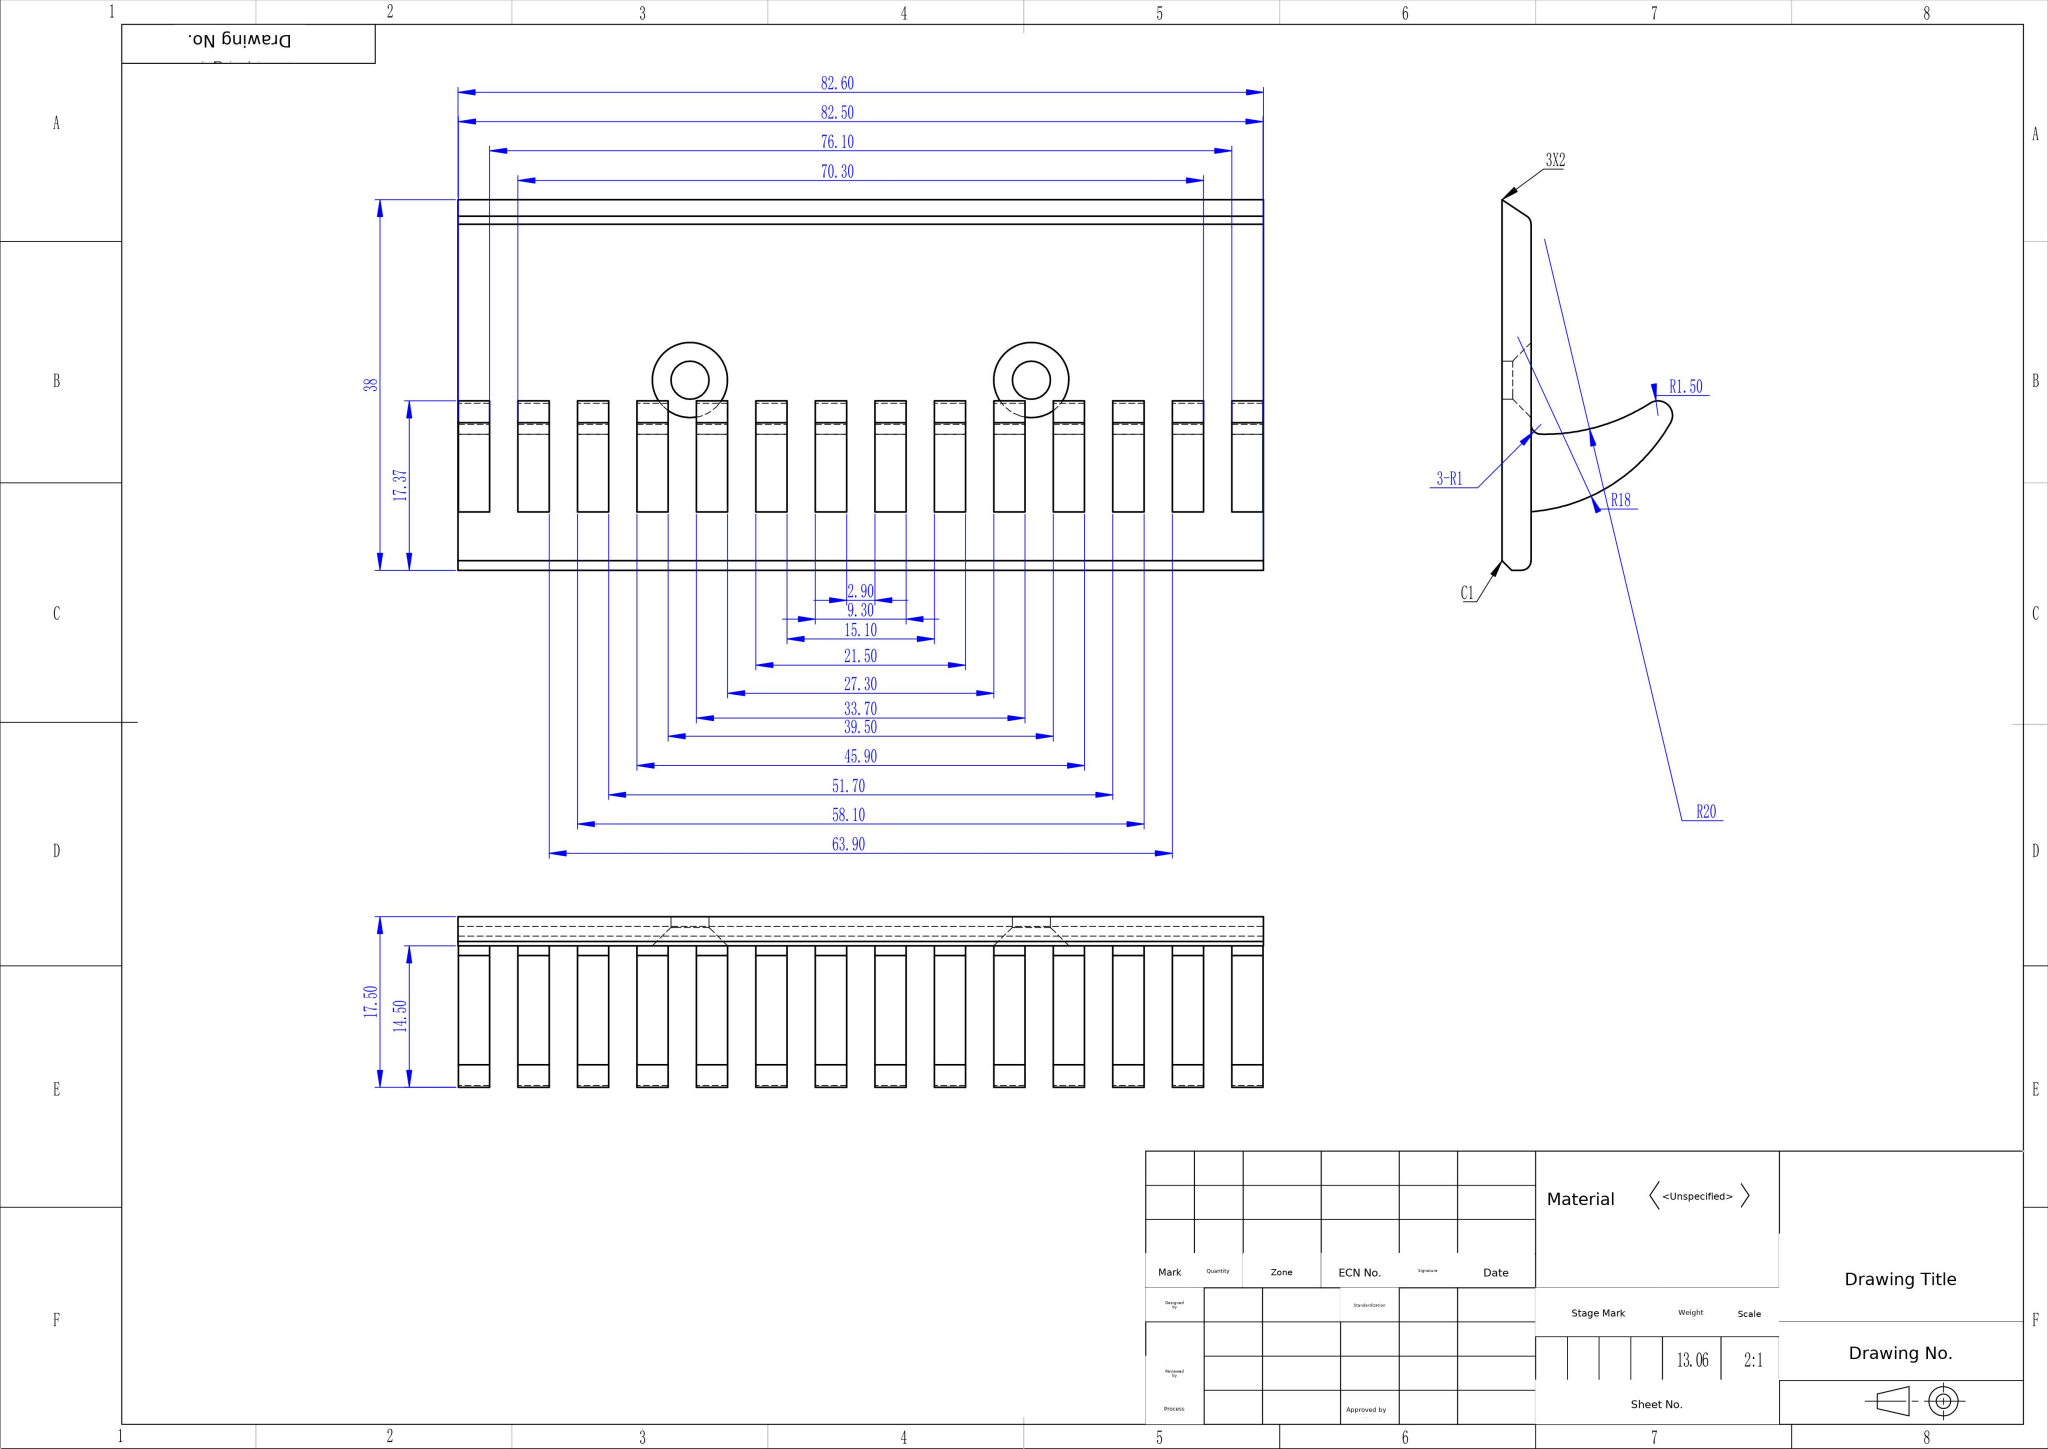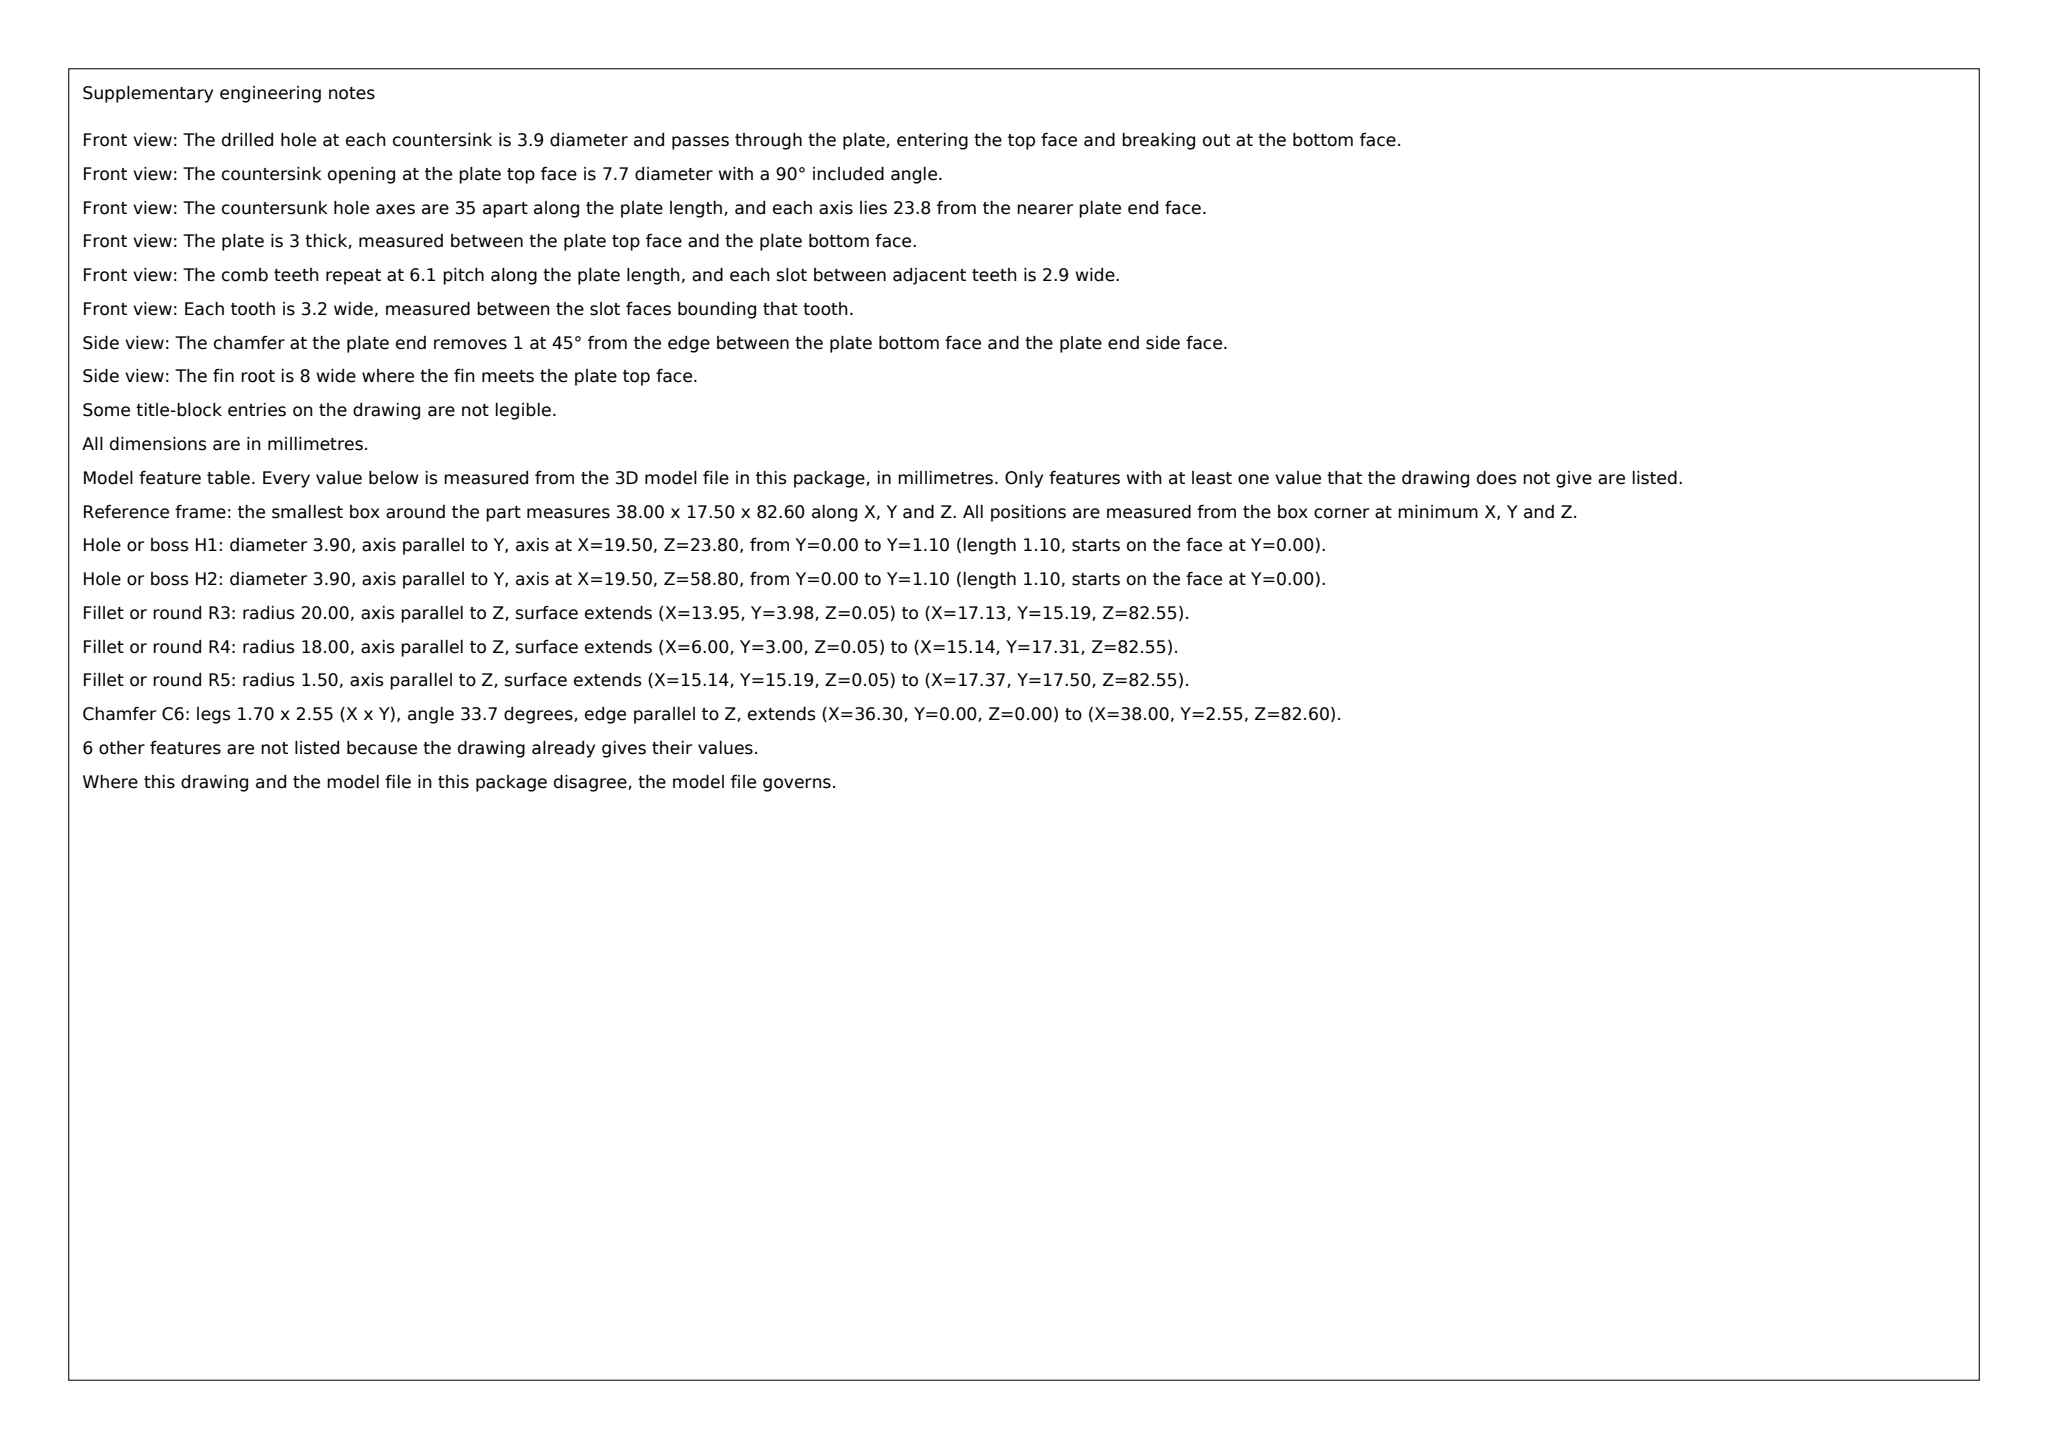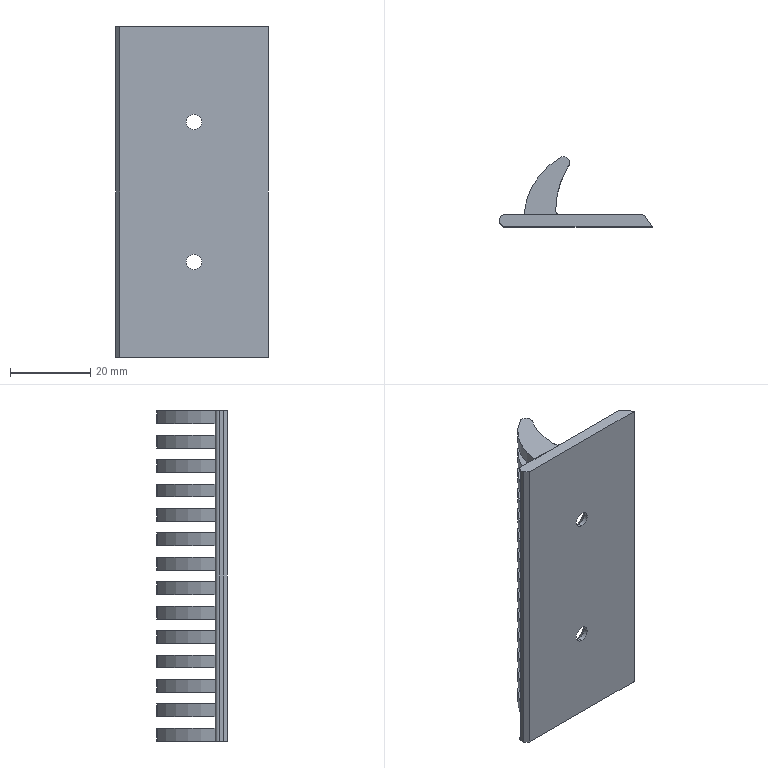Part | SolidWorks | mm | 1 solid | 115 faces | box 38 x 17.5 x 82.6 mm | volume 13060 mm3 | cylinder 76 | plane 35 | cone 4 | commonest cylinder face diameters 40 x28 2 x16 3 x14 36 x14 3.9 x4
Drawing notes:
SIDE VIEW: R18 CTR 23.95 FROM BOT EDGE, 1.61 FROM BACK FACE | from the solid: cyl dia 36.0 axis z at (x=23.95, y=1.61), len 3.2 x14
SIDE VIEW: R20 CTR 33.95 FROM BOT EDGE, 4.37 FROM BACK FACE | from the solid: cyl dia 40.0 axis z at (x=33.95, y=4.37), len 3.2 x28
R1.50 TIP CTR 15.87 FROM BOT EDGE, 16.00 FROM BACK FACE | from the solid: cyl dia 3.0 axis z at (x=15.87, y=16.0), len 3.2 x14; tangent to bbox y=17.5 and x=17.37
3-R1 CTRS 1.00, 14.96 & 35.46 FROM BOT EDGE, TANG 3.00 FACE | from the solid: cyl dia 2.0 at (1.00,2.00) L82.6, (35.46,2.00) L82.6, (14.96,4.00) L3.2 x14
TOP EDGE, SIDE VIEW: CHAMFER 3 X 2 (3 DOWN X 2 ACROSS 3 THK WALL) | from the solid: Side-view wall bounded by y-planes 0.0 and 3.0 (3 THK); top edge of 38 x 82.6 plate cut back, matching 3X2 leader; no fillet radii listed
build123d program:
from build123d import *

# Parameters (mm, degrees)
SKETCH3_W                                    = 25
SKETCH3_H                                    = 3
BOSS_EXTRUDE2_DEPTH                          = 82.6
BOSS_EXTRUDE3_DEPTH                          = 82.6
FILLET3_R                                    = 1
BOSS_EXTRUDE4_DEPTH                          = 82.6
SKETCH9_W                                    = 6
SKETCH9_H                                    = 3
BOSS_EXTRUDE5_DEPTH                          = 82.6
CHAMFER1_SIZE                                = 1
FILLET1_R                                    = 1
CONICAL_COUNTERSUNK_HOLE_FOR_M3_5_PH_2_COUNT = 2
CONICAL_COUNTERSUNK_HOLE_FOR_M3_5_PH_2_PITCH = 35
SKETCH12_W                                   = 42.466
SKETCH12_H                                   = 2.9
CUT_EXTRUDE1_DEPTH                           = 90.761
LPATTERN1_COUNT                              = 22
LPATTERN1_PITCH                              = 6.1
MIRROR1_COPY_1_SKETCH_W                      = 42.466
MIRROR1_COPY_1_SKETCH_H                      = 2.9
MIRROR1_COPY_1_DEPTH                         = 90.761
MIRROR1_COPY_2_SKETCH_W                      = 42.466
MIRROR1_COPY_2_SKETCH_H                      = 2.9
MIRROR1_COPY_2_DEPTH                         = 90.761
MIRROR1_COPY_3_SKETCH_W                      = 42.466
MIRROR1_COPY_3_SKETCH_H                      = 2.9
MIRROR1_COPY_3_DEPTH                         = 90.761
MIRROR1_COPY_4_SKETCH_W                      = 42.466
MIRROR1_COPY_4_SKETCH_H                      = 2.9
MIRROR1_COPY_4_DEPTH                         = 90.761
MIRROR1_COPY_5_SKETCH_W                      = 42.466
MIRROR1_COPY_5_SKETCH_H                      = 2.9
MIRROR1_COPY_5_DEPTH                         = 90.761
MIRROR1_COPY_6_SKETCH_W                      = 42.466
MIRROR1_COPY_6_SKETCH_H                      = 2.9
MIRROR1_COPY_6_DEPTH                         = 90.761
MIRROR1_COPY_7_SKETCH_W                      = 42.466
MIRROR1_COPY_7_SKETCH_H                      = 2.9
MIRROR1_COPY_7_DEPTH                         = 90.761
MIRROR1_COPY_8_SKETCH_W                      = 42.466
MIRROR1_COPY_8_SKETCH_H                      = 2.9
MIRROR1_COPY_8_DEPTH                         = 90.761
MIRROR1_COPY_9_SKETCH_W                      = 42.466
MIRROR1_COPY_9_SKETCH_H                      = 2.9
MIRROR1_COPY_9_DEPTH                         = 90.761
MIRROR1_COPY_10_SKETCH_W                     = 42.466
MIRROR1_COPY_10_SKETCH_H                     = 2.9
MIRROR1_COPY_10_DEPTH                        = 90.761
MIRROR1_COPY_11_SKETCH_W                     = 42.466
MIRROR1_COPY_11_SKETCH_H                     = 2.9
MIRROR1_COPY_11_DEPTH                        = 90.761
MIRROR1_COPY_12_SKETCH_W                     = 42.466
MIRROR1_COPY_12_SKETCH_H                     = 2.9
MIRROR1_COPY_12_DEPTH                        = 90.761
MIRROR1_COPY_13_SKETCH_W                     = 42.466
MIRROR1_COPY_13_SKETCH_H                     = 2.9
MIRROR1_COPY_13_DEPTH                        = 90.761
MIRROR1_COPY_14_SKETCH_W                     = 42.466
MIRROR1_COPY_14_SKETCH_H                     = 2.9
MIRROR1_COPY_14_DEPTH                        = 90.761
MIRROR1_COPY_15_SKETCH_W                     = 42.466
MIRROR1_COPY_15_SKETCH_H                     = 2.9
MIRROR1_COPY_15_DEPTH                        = 90.761
MIRROR1_COPY_16_SKETCH_W                     = 42.466
MIRROR1_COPY_16_SKETCH_H                     = 2.9
MIRROR1_COPY_16_DEPTH                        = 90.761
MIRROR1_COPY_17_SKETCH_W                     = 42.466
MIRROR1_COPY_17_SKETCH_H                     = 2.9
MIRROR1_COPY_17_DEPTH                        = 90.761
MIRROR1_COPY_18_SKETCH_W                     = 42.466
MIRROR1_COPY_18_SKETCH_H                     = 2.9
MIRROR1_COPY_18_DEPTH                        = 90.761
MIRROR1_COPY_19_SKETCH_W                     = 42.466
MIRROR1_COPY_19_SKETCH_H                     = 2.9
MIRROR1_COPY_19_DEPTH                        = 90.761
MIRROR1_COPY_20_SKETCH_W                     = 42.466
MIRROR1_COPY_20_SKETCH_H                     = 2.9
MIRROR1_COPY_20_DEPTH                        = 90.761
MIRROR1_COPY_21_SKETCH_W                     = 42.466
MIRROR1_COPY_21_SKETCH_H                     = 2.9
MIRROR1_COPY_21_DEPTH                        = 90.761
MIRROR1_COPY_22_SKETCH_W                     = 42.466
MIRROR1_COPY_22_SKETCH_H                     = 2.9
MIRROR1_COPY_22_DEPTH                        = 90.761


with BuildPart() as part:
    # Sketch3 → Boss-Extrude2 (new body)
    with BuildSketch(Plane.XY):
        with Locations((12.5, -1.5)):
            Rectangle(SKETCH3_W, SKETCH3_H)
    extrude(amount=BOSS_EXTRUDE2_DEPTH)

    # Sketch4 → Boss-Extrude3 (add)
    with BuildSketch(Plane(origin=(0, 0, 0), x_dir=(-1, 0, 0), z_dir=(0, 0, -1))):
        with BuildLine():
            Line((0, 0), (-8, 0))
            ThreePointArc((-8, 0), (-8.582, 6.347), (-11.132, 12.189))
            ThreePointArc((-11.132, 12.189), (-10.962, 14.028), (-9.136, 14.308))
            ThreePointArc((-9.136, 14.308), (-2.775, 8.299), (0, 0))
        make_face()
    extrude(amount=-BOSS_EXTRUDE3_DEPTH)

    # Fillet3
    fillet3_edges = [part.edges().sort_by_distance(p)[0] for p in [
        (8, 0, 41.3),
    ]]
    fillet(fillet3_edges, radius=FILLET3_R)

    # Sketch8 → Boss-Extrude4 (add)
    with BuildSketch(Plane.XY.offset(82.6)):
        with BuildLine():
            Line((32, -3), (25, -3))
            Line((25, -3), (25, 0))
            Line((25, 0), (29.465, 0))
            ThreePointArc((29.465, 0), (29.937, -0.1183), (30.297, -0.4453))
            Line((30.297, -0.4453), (32, -3))
        make_face()
    extrude(amount=-BOSS_EXTRUDE4_DEPTH)

    # Sketch9 → Boss-Extrude5 (add)
    with BuildSketch(Plane.XY.offset(82.6)):
        with Locations((-3, -1.5)):
            Rectangle(SKETCH9_W, SKETCH9_H)
    extrude(amount=-BOSS_EXTRUDE5_DEPTH)

    # Chamfer1
    chamfer1_edges = [part.edges().sort_by_distance(p)[0] for p in [
        (-6, -3, 41.3),
    ]]
    chamfer(chamfer1_edges, length=CHAMFER1_SIZE)

    # Fillet1
    fillet1_edges = [part.edges().sort_by_distance(p)[0] for p in [
        (-6, 0, 41.3),
    ]]
    fillet(fillet1_edges, radius=FILLET1_R)

    # Sketch11 → Conical Countersunk Hole for M3.5 Philli (revolve, cut)
    with BuildSketch(Plane(origin=(13.5, 0, 23.8), x_dir=(0, 0, 1), z_dir=(1, 0, 0))):
        Polygon((0, 0), (0, 3), (1.95, 3), (1.95, 1.9), (3.85, 0), align=None)
    conical_countersunk_hole_for_m3_5_philli = revolve(axis=Axis((13.5, 6.35, 23.8), (0, -1, 0)), mode=Mode.SUBTRACT)

    # Conical Countersunk Hole for M3.5 Ph 2: Conical Countersunk Hole for M3.5 Philli ×2
    with Locations(*[(0, 0, i * CONICAL_COUNTERSUNK_HOLE_FOR_M3_5_PH_2_PITCH) for i in range(1, CONICAL_COUNTERSUNK_HOLE_FOR_M3_5_PH_2_COUNT)]):
        add(conical_countersunk_hole_for_m3_5_philli, mode=Mode.SUBTRACT)

    # Sketch12 → Cut-Extrude1 (cut, through all)
    with BuildSketch(Plane(origin=(0, 0, 0), x_dir=(1, 0, 0), z_dir=(0, 1, 0))):
        with Locations((11.808, -41.3)):
            Rectangle(SKETCH12_W, SKETCH12_H)
    cut_extrude1 = extrude(amount=CUT_EXTRUDE1_DEPTH, mode=Mode.SUBTRACT)

    # LPattern1: Cut-Extrude1 ×22
    with Locations(*[(0, 0, i * LPATTERN1_PITCH) for i in range(1, LPATTERN1_COUNT)]):
        add(cut_extrude1, mode=Mode.SUBTRACT)

    # Mirror1 copy 1 sketch → Mirror1 copy 1 (cut, through all)
    with BuildSketch(Plane(origin=(0, 0, 76.5), x_dir=(1, 0, 0), z_dir=(0, 1, 0))):
        with Locations((11.808, 41.3)):
            Rectangle(MIRROR1_COPY_1_SKETCH_W, MIRROR1_COPY_1_SKETCH_H)
    extrude(amount=MIRROR1_COPY_1_DEPTH, mode=Mode.SUBTRACT)

    # Mirror1 copy 2 sketch → Mirror1 copy 2 (cut, through all)
    with BuildSketch(Plane(origin=(0, 0, 70.4), x_dir=(1, 0, 0), z_dir=(0, 1, 0))):
        with Locations((11.808, 41.3)):
            Rectangle(MIRROR1_COPY_2_SKETCH_W, MIRROR1_COPY_2_SKETCH_H)
    extrude(amount=MIRROR1_COPY_2_DEPTH, mode=Mode.SUBTRACT)

    # Mirror1 copy 3 sketch → Mirror1 copy 3 (cut, through all)
    with BuildSketch(Plane(origin=(0, 0, 64.3), x_dir=(1, 0, 0), z_dir=(0, 1, 0))):
        with Locations((11.808, 41.3)):
            Rectangle(MIRROR1_COPY_3_SKETCH_W, MIRROR1_COPY_3_SKETCH_H)
    extrude(amount=MIRROR1_COPY_3_DEPTH, mode=Mode.SUBTRACT)

    # Mirror1 copy 4 sketch → Mirror1 copy 4 (cut, through all)
    with BuildSketch(Plane(origin=(0, 0, 58.2), x_dir=(1, 0, 0), z_dir=(0, 1, 0))):
        with Locations((11.808, 41.3)):
            Rectangle(MIRROR1_COPY_4_SKETCH_W, MIRROR1_COPY_4_SKETCH_H)
    extrude(amount=MIRROR1_COPY_4_DEPTH, mode=Mode.SUBTRACT)

    # Mirror1 copy 5 sketch → Mirror1 copy 5 (cut, through all)
    with BuildSketch(Plane(origin=(0, 0, 52.1), x_dir=(1, 0, 0), z_dir=(0, 1, 0))):
        with Locations((11.808, 41.3)):
            Rectangle(MIRROR1_COPY_5_SKETCH_W, MIRROR1_COPY_5_SKETCH_H)
    extrude(amount=MIRROR1_COPY_5_DEPTH, mode=Mode.SUBTRACT)

    # Mirror1 copy 6 sketch → Mirror1 copy 6 (cut, through all)
    with BuildSketch(Plane(origin=(0, 0, 46), x_dir=(1, 0, 0), z_dir=(0, 1, 0))):
        with Locations((11.808, 41.3)):
            Rectangle(MIRROR1_COPY_6_SKETCH_W, MIRROR1_COPY_6_SKETCH_H)
    extrude(amount=MIRROR1_COPY_6_DEPTH, mode=Mode.SUBTRACT)

    # Mirror1 copy 7 sketch → Mirror1 copy 7 (cut, through all)
    with BuildSketch(Plane(origin=(0, 0, 39.9), x_dir=(1, 0, 0), z_dir=(0, 1, 0))):
        with Locations((11.808, 41.3)):
            Rectangle(MIRROR1_COPY_7_SKETCH_W, MIRROR1_COPY_7_SKETCH_H)
    extrude(amount=MIRROR1_COPY_7_DEPTH, mode=Mode.SUBTRACT)

    # Mirror1 copy 8 sketch → Mirror1 copy 8 (cut, through all)
    with BuildSketch(Plane(origin=(0, 0, 33.8), x_dir=(1, 0, 0), z_dir=(0, 1, 0))):
        with Locations((11.808, 41.3)):
            Rectangle(MIRROR1_COPY_8_SKETCH_W, MIRROR1_COPY_8_SKETCH_H)
    extrude(amount=MIRROR1_COPY_8_DEPTH, mode=Mode.SUBTRACT)

    # Mirror1 copy 9 sketch → Mirror1 copy 9 (cut, through all)
    with BuildSketch(Plane(origin=(0, 0, 27.7), x_dir=(1, 0, 0), z_dir=(0, 1, 0))):
        with Locations((11.808, 41.3)):
            Rectangle(MIRROR1_COPY_9_SKETCH_W, MIRROR1_COPY_9_SKETCH_H)
    extrude(amount=MIRROR1_COPY_9_DEPTH, mode=Mode.SUBTRACT)

    # Mirror1 copy 10 sketch → Mirror1 copy 10 (cut, through all)
    with BuildSketch(Plane(origin=(0, 0, 21.6), x_dir=(1, 0, 0), z_dir=(0, 1, 0))):
        with Locations((11.808, 41.3)):
            Rectangle(MIRROR1_COPY_10_SKETCH_W, MIRROR1_COPY_10_SKETCH_H)
    extrude(amount=MIRROR1_COPY_10_DEPTH, mode=Mode.SUBTRACT)

    # Mirror1 copy 11 sketch → Mirror1 copy 11 (cut, through all)
    with BuildSketch(Plane(origin=(0, 0, 15.5), x_dir=(1, 0, 0), z_dir=(0, 1, 0))):
        with Locations((11.808, 41.3)):
            Rectangle(MIRROR1_COPY_11_SKETCH_W, MIRROR1_COPY_11_SKETCH_H)
    extrude(amount=MIRROR1_COPY_11_DEPTH, mode=Mode.SUBTRACT)

    # Mirror1 copy 12 sketch → Mirror1 copy 12 (cut, through all)
    with BuildSketch(Plane(origin=(0, 0, 9.4), x_dir=(1, 0, 0), z_dir=(0, 1, 0))):
        with Locations((11.808, 41.3)):
            Rectangle(MIRROR1_COPY_12_SKETCH_W, MIRROR1_COPY_12_SKETCH_H)
    extrude(amount=MIRROR1_COPY_12_DEPTH, mode=Mode.SUBTRACT)

    # Mirror1 copy 13 sketch → Mirror1 copy 13 (cut, through all)
    with BuildSketch(Plane(origin=(0, 0, 3.3), x_dir=(1, 0, 0), z_dir=(0, 1, 0))):
        with Locations((11.808, 41.3)):
            Rectangle(MIRROR1_COPY_13_SKETCH_W, MIRROR1_COPY_13_SKETCH_H)
    extrude(amount=MIRROR1_COPY_13_DEPTH, mode=Mode.SUBTRACT)

    # Mirror1 copy 14 sketch → Mirror1 copy 14 (cut, through all)
    with BuildSketch(Plane(origin=(0, 0, -2.8), x_dir=(1, 0, 0), z_dir=(0, 1, 0))):
        with Locations((11.808, 41.3)):
            Rectangle(MIRROR1_COPY_14_SKETCH_W, MIRROR1_COPY_14_SKETCH_H)
    extrude(amount=MIRROR1_COPY_14_DEPTH, mode=Mode.SUBTRACT)

    # Mirror1 copy 15 sketch → Mirror1 copy 15 (cut, through all)
    with BuildSketch(Plane(origin=(0, 0, -8.9), x_dir=(1, 0, 0), z_dir=(0, 1, 0))):
        with Locations((11.808, 41.3)):
            Rectangle(MIRROR1_COPY_15_SKETCH_W, MIRROR1_COPY_15_SKETCH_H)
    extrude(amount=MIRROR1_COPY_15_DEPTH, mode=Mode.SUBTRACT)

    # Mirror1 copy 16 sketch → Mirror1 copy 16 (cut, through all)
    with BuildSketch(Plane(origin=(0, 0, -15), x_dir=(1, 0, 0), z_dir=(0, 1, 0))):
        with Locations((11.808, 41.3)):
            Rectangle(MIRROR1_COPY_16_SKETCH_W, MIRROR1_COPY_16_SKETCH_H)
    extrude(amount=MIRROR1_COPY_16_DEPTH, mode=Mode.SUBTRACT)

    # Mirror1 copy 17 sketch → Mirror1 copy 17 (cut, through all)
    with BuildSketch(Plane(origin=(0, 0, -21.1), x_dir=(1, 0, 0), z_dir=(0, 1, 0))):
        with Locations((11.808, 41.3)):
            Rectangle(MIRROR1_COPY_17_SKETCH_W, MIRROR1_COPY_17_SKETCH_H)
    extrude(amount=MIRROR1_COPY_17_DEPTH, mode=Mode.SUBTRACT)

    # Mirror1 copy 18 sketch → Mirror1 copy 18 (cut, through all)
    with BuildSketch(Plane(origin=(0, 0, -27.2), x_dir=(1, 0, 0), z_dir=(0, 1, 0))):
        with Locations((11.808, 41.3)):
            Rectangle(MIRROR1_COPY_18_SKETCH_W, MIRROR1_COPY_18_SKETCH_H)
    extrude(amount=MIRROR1_COPY_18_DEPTH, mode=Mode.SUBTRACT)

    # Mirror1 copy 19 sketch → Mirror1 copy 19 (cut, through all)
    with BuildSketch(Plane(origin=(0, 0, -33.3), x_dir=(1, 0, 0), z_dir=(0, 1, 0))):
        with Locations((11.808, 41.3)):
            Rectangle(MIRROR1_COPY_19_SKETCH_W, MIRROR1_COPY_19_SKETCH_H)
    extrude(amount=MIRROR1_COPY_19_DEPTH, mode=Mode.SUBTRACT)

    # Mirror1 copy 20 sketch → Mirror1 copy 20 (cut, through all)
    with BuildSketch(Plane(origin=(0, 0, -39.4), x_dir=(1, 0, 0), z_dir=(0, 1, 0))):
        with Locations((11.808, 41.3)):
            Rectangle(MIRROR1_COPY_20_SKETCH_W, MIRROR1_COPY_20_SKETCH_H)
    extrude(amount=MIRROR1_COPY_20_DEPTH, mode=Mode.SUBTRACT)

    # Mirror1 copy 21 sketch → Mirror1 copy 21 (cut, through all)
    with BuildSketch(Plane(origin=(0, 0, -45.5), x_dir=(1, 0, 0), z_dir=(0, 1, 0))):
        with Locations((11.808, 41.3)):
            Rectangle(MIRROR1_COPY_21_SKETCH_W, MIRROR1_COPY_21_SKETCH_H)
    extrude(amount=MIRROR1_COPY_21_DEPTH, mode=Mode.SUBTRACT)

    # Mirror1 copy 22 sketch → Mirror1 copy 22 (cut, through all)
    with BuildSketch(Plane(origin=(0, 0, 82.6), x_dir=(1, 0, 0), z_dir=(0, 1, 0))):
        with Locations((11.808, 41.3)):
            Rectangle(MIRROR1_COPY_22_SKETCH_W, MIRROR1_COPY_22_SKETCH_H)
    extrude(amount=MIRROR1_COPY_22_DEPTH, mode=Mode.SUBTRACT)


solid = part.part